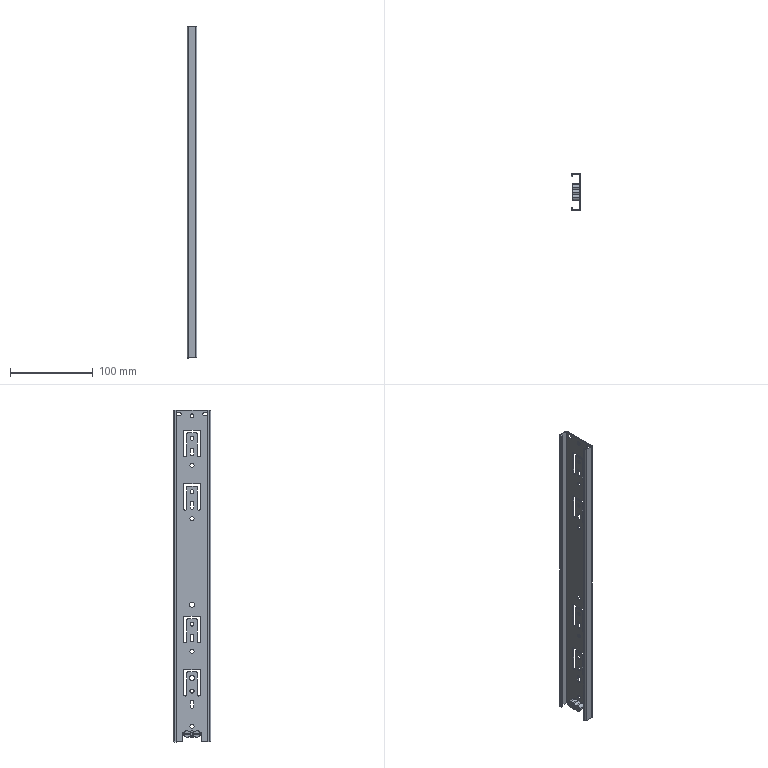Component | SolidWorks | PC-CAJ-P08-1_Corredera A 400-1 | 1 solid | 173 faces | volume 32228 mm3 | plane 91 | cylinder 82 | commonest cylinder face diameters 2 x16 4.7 x15 5 x10 8 x9 3.8 x8 1 x5 3.4 x5 4.6 x3 | material Plain Carbon Steel